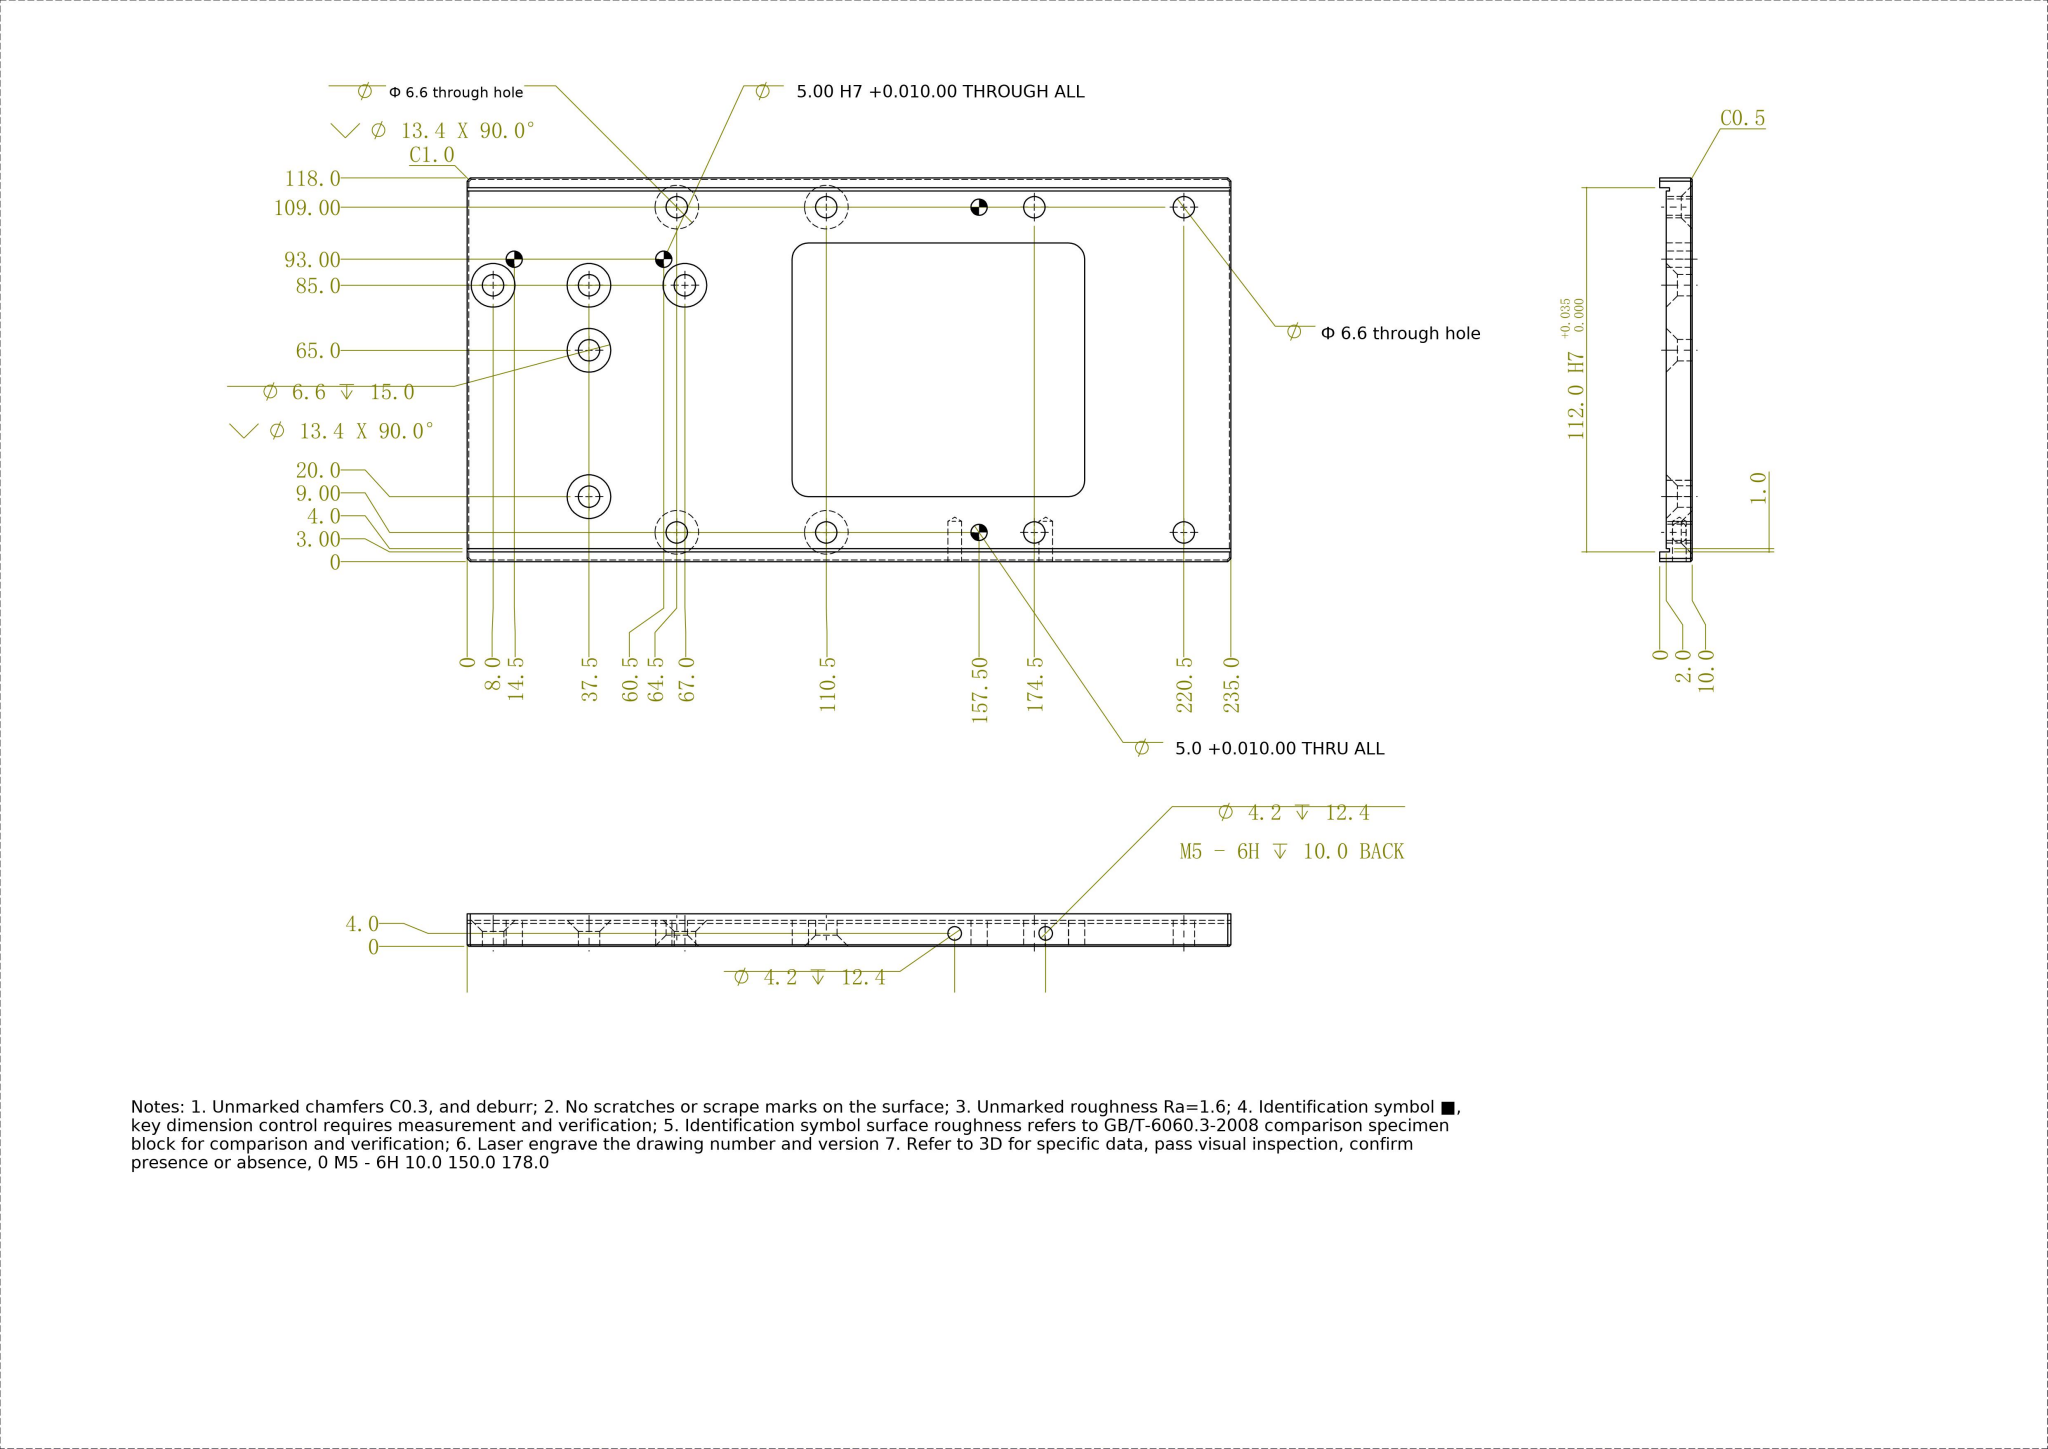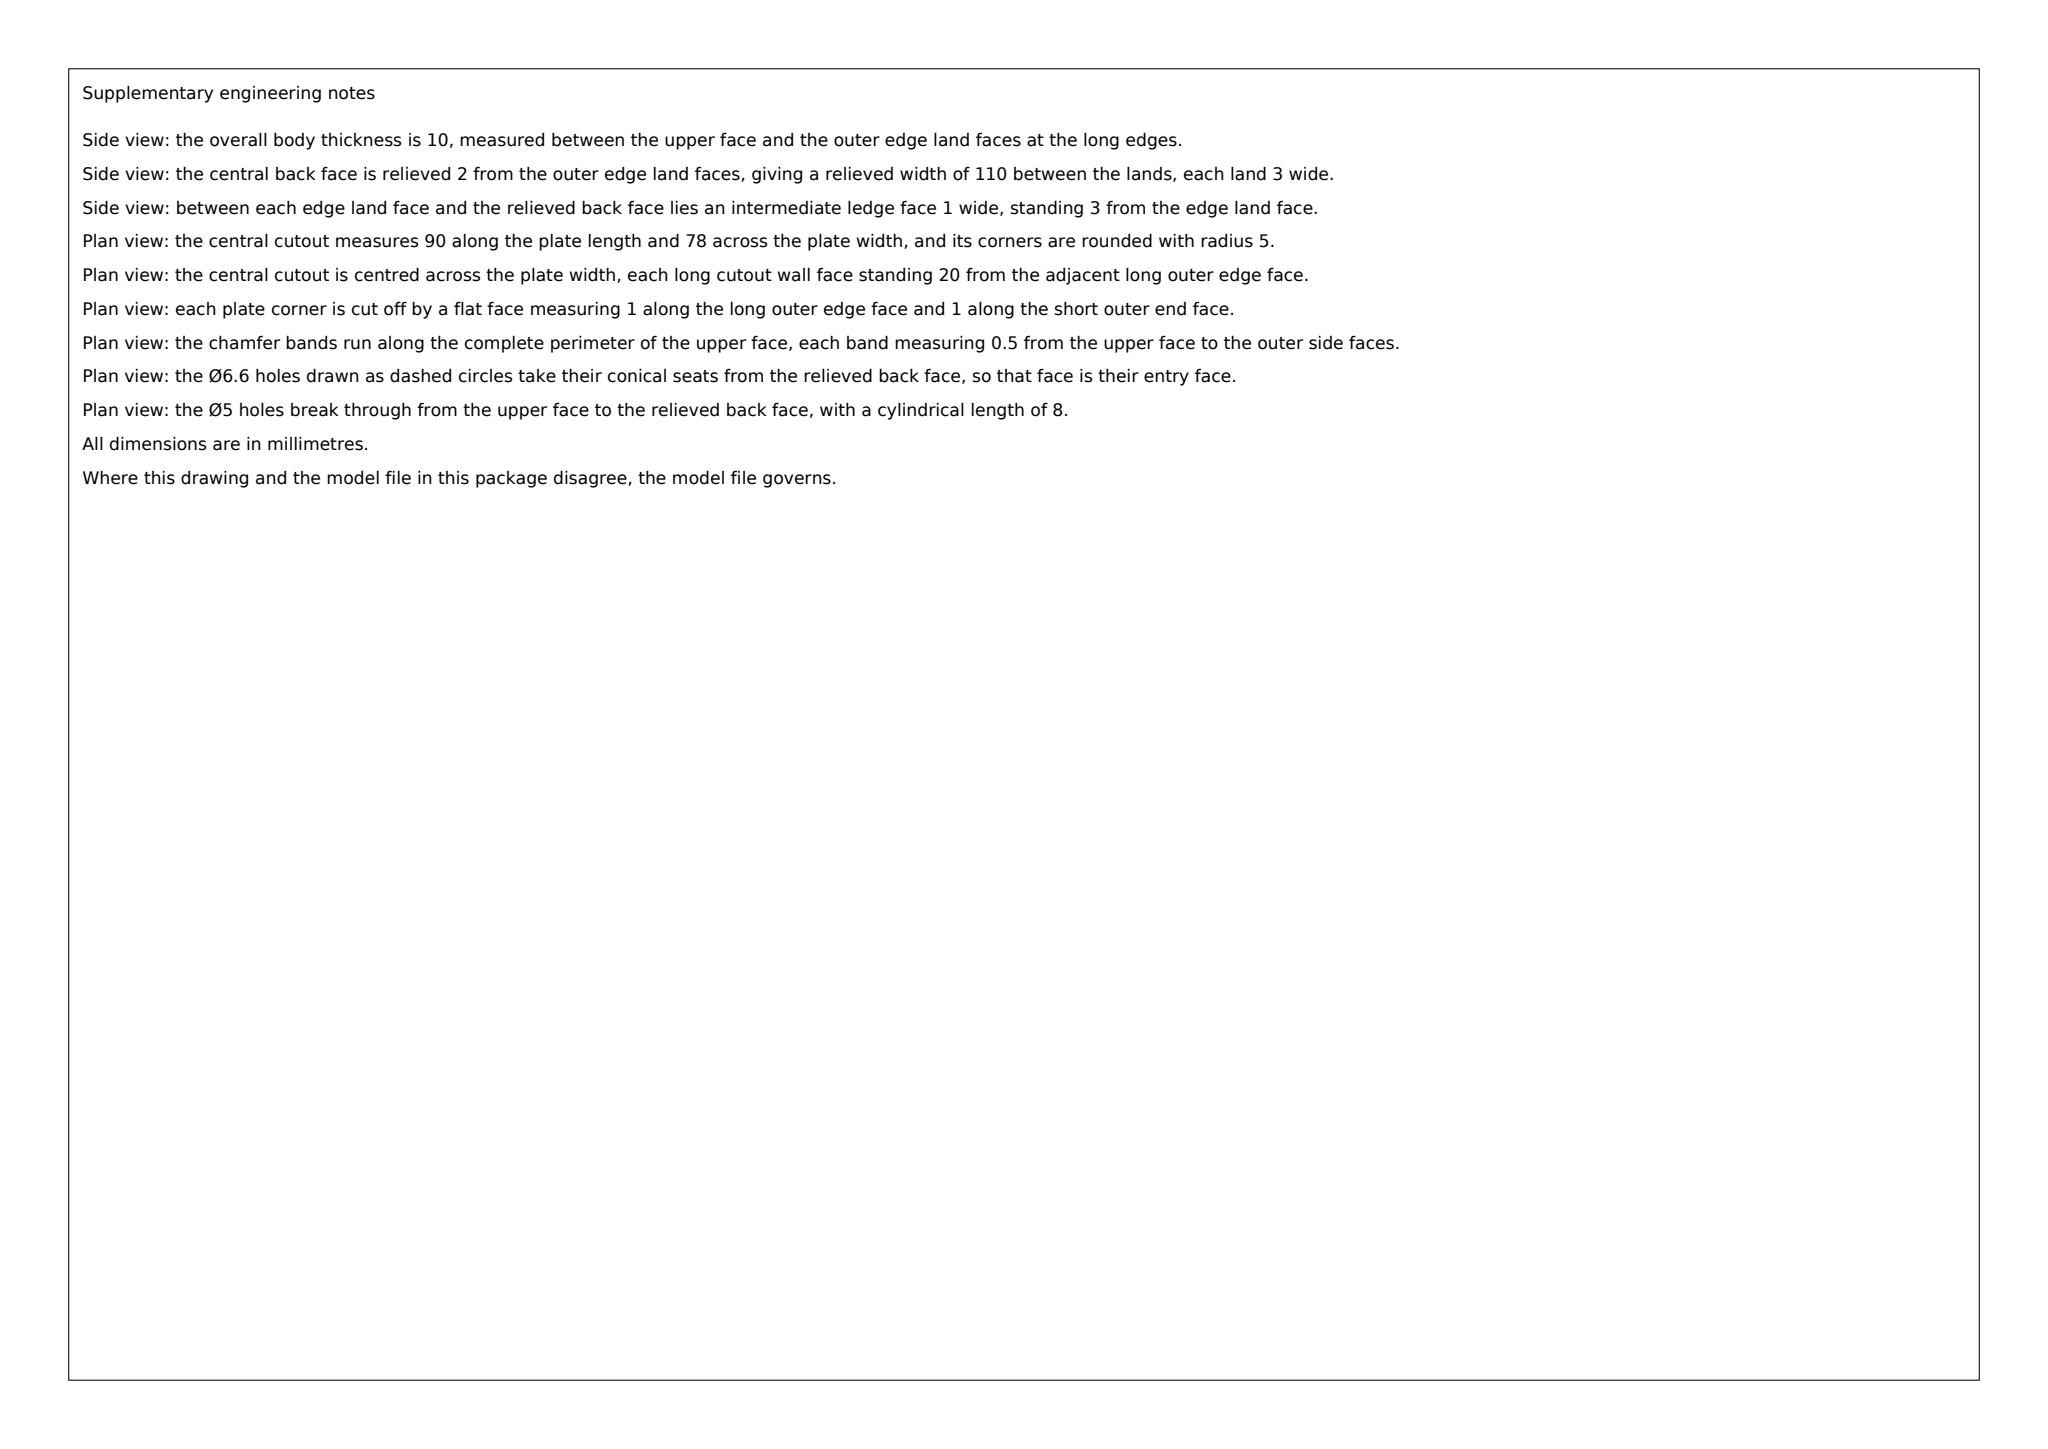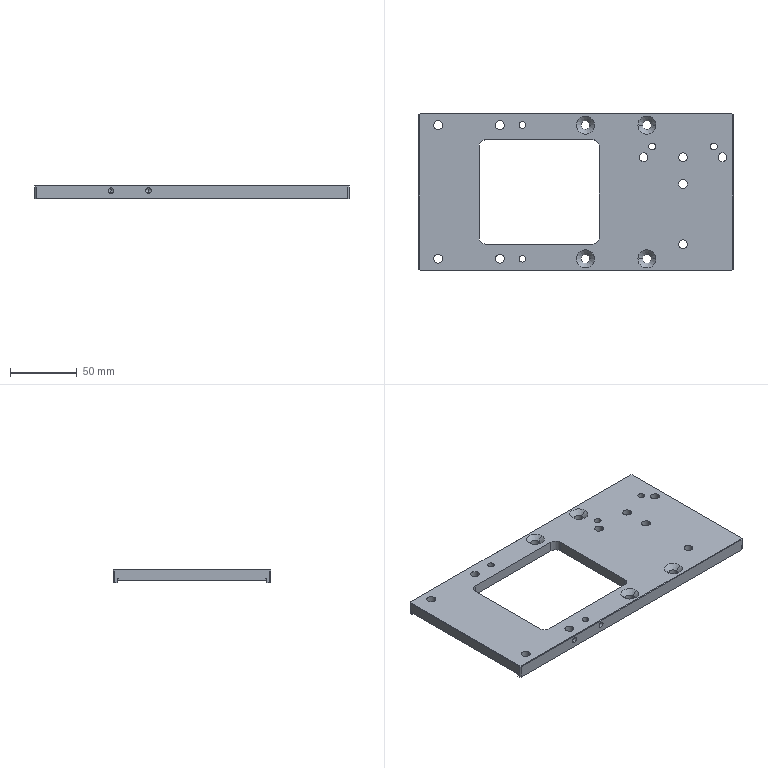Part | SolidWorks | mm | 1 solid | 94 faces | box 235 x 118 x 10 mm | volume 162108 mm3 | cylinder 42 | plane 30 | cone 22 | commonest cylinder face diameters 6.6 x26 5 x8 4.2 x4 10 x4
Drawing notes:
STOCK 235.0 X 118.0 X 10.0 THK | from the solid: bbox_xyz 235.0 x 118.0 x 10.0
CTR POCKET 90.0 W X 78.0 H DP 8.0, R5.0 CNRS, LOC 100.0 & 20.0 | from the solid: x-planes 45.0/135.0 = 90 wide (drawing 100.0-190.0); y-planes 20.0/98.0 = 78 high; floor z=2.0 in 10.0 thk = DP 8.0; 4X R5 cnrs
2X M5-6H DP 10.0, Ø4.2 DP 12.4 IN BACK EDGE AT 150.0/178.0, 6.0 FR BTM | from the solid: cyl Ø4.2 axis y at x=57.0 & 85.0 (=235-178.0 / 235-150.0), z=6.0, length 12.4; cone 118° ref dia 4.2 drill point